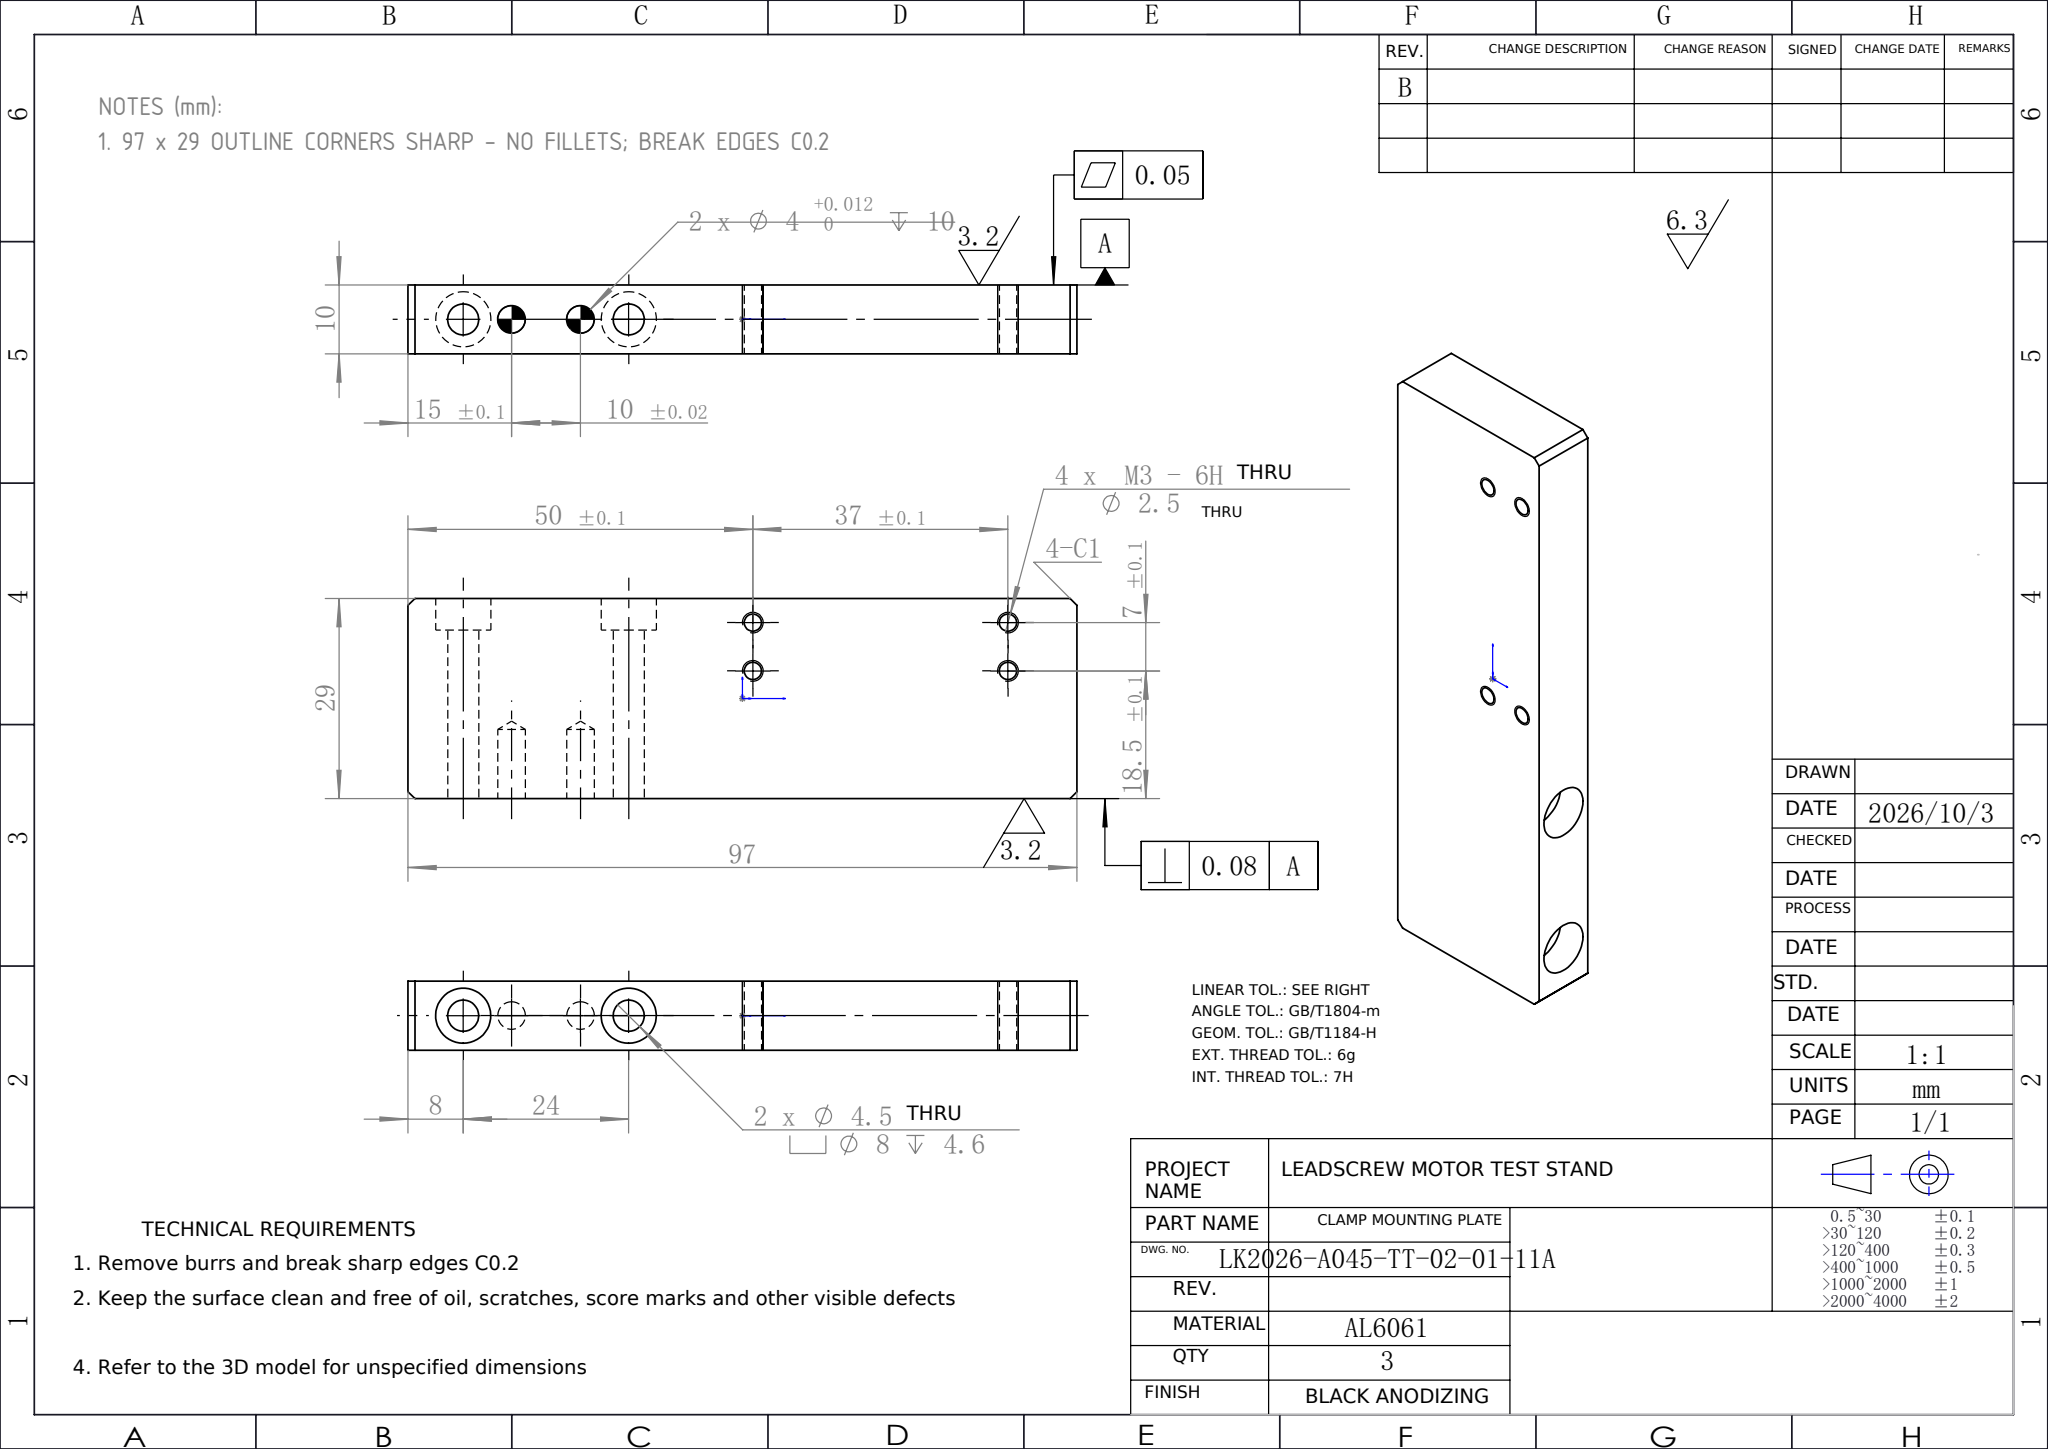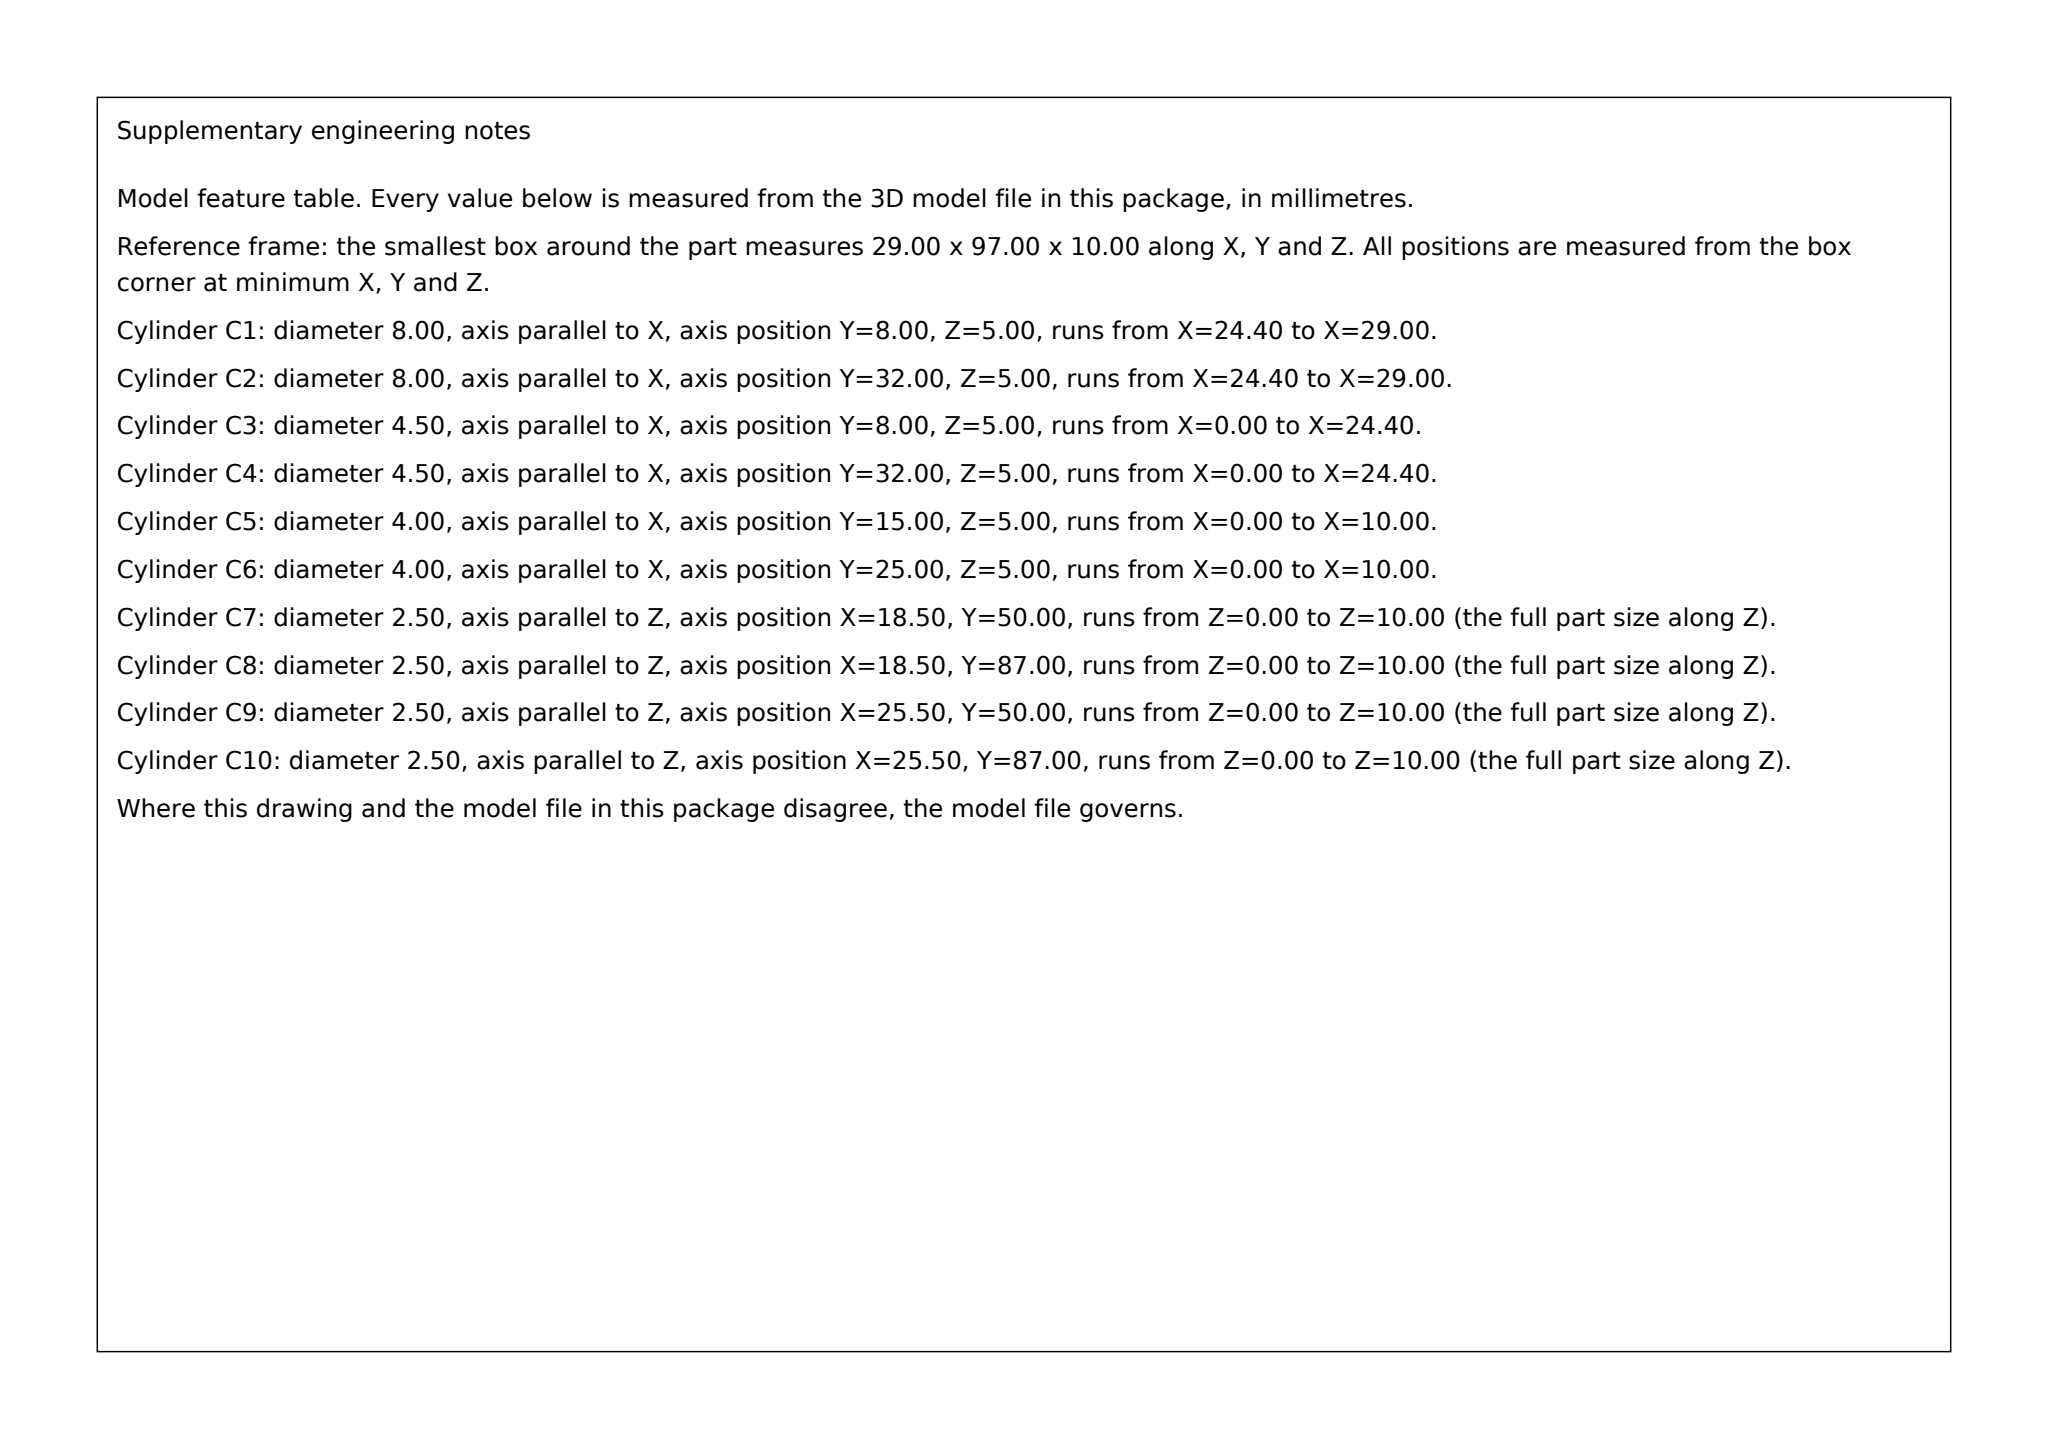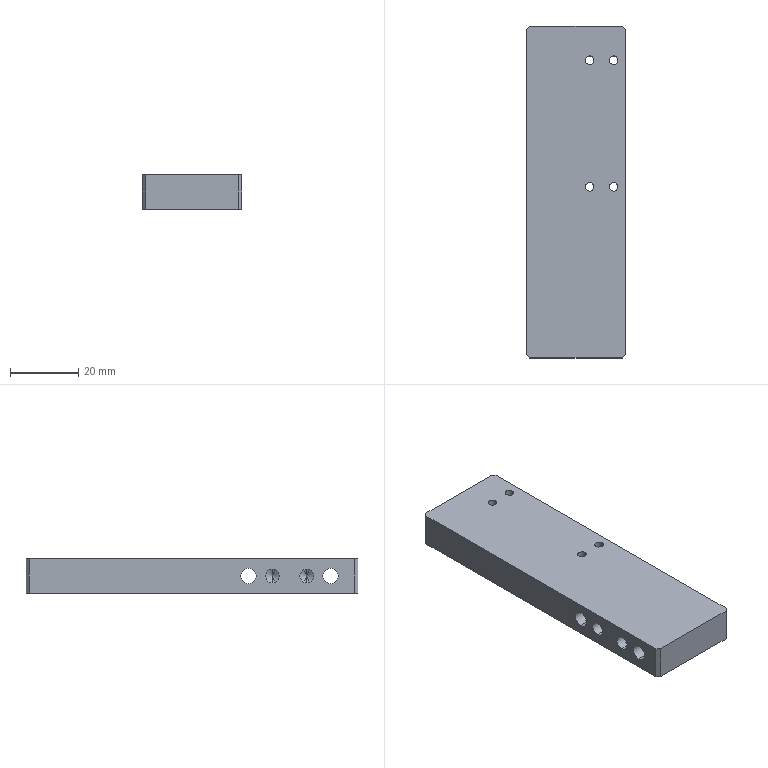Part | SolidWorks | mm | 1 solid | 36 faces | box 29 x 97 x 10 mm | volume 26414 mm3 | cylinder 20 | plane 12 | cone 4 | commonest cylinder face diameters 2.5 x8 4 x4 8 x4 4.5 x4
Drawing notes:
97 x 29 OUTLINE CORNERS SHARP - NO FILLETS; BREAK EDGES C0.2 | from the solid: fillet_radii: []; planar faces x=0/29.0, y=0/97.0; bbox 29.0 x 97.0 x 10.0
build123d program:
from build123d import *

# Parameters (mm, degrees)
SKETCH1_W                                       = 29
SKETCH1_H                                       = 97
BOSS_EXTRUDE1_DEPTH                             = 5
M4_HEX_SOCKET_HEAD_CAP_SCREW_CBORE1_D           = 4.5
M4_HEX_SOCKET_HEAD_CAP_SCREW_CBORE1_CBORE_D     = 8
M4_HEX_SOCKET_HEAD_CAP_SCREW_CBORE1_CBORE_DEPTH = 4.6
F_4_0MM_DOWEL_PIN_HOLE1_D                       = 4
F_4_0MM_DOWEL_PIN_HOLE1_DEPTH                   = 10
F_4_0MM_DOWEL_PIN_HOLE1_TIP                     = 1.202
M3_TAPPED_HOLE1_D                               = 2.5
CHAMFER1_SIZE                                   = 1


with BuildPart() as part:
    # Sketch1 → Boss-Extrude1 (new, symmetric)
    with BuildSketch(Plane.XY):
        Rectangle(SKETCH1_W, SKETCH1_H)
    extrude(amount=BOSS_EXTRUDE1_DEPTH, both=True)

    # M4 Hex Socket Head Cap Screw CBORE1 (through all)
    with Locations(Plane(origin=(14.5, 0, 0), x_dir=(0, 0, -1), z_dir=(1, 0, 0))):
        with Locations((0, -40.5), (0, -16.5)):
            CounterBoreHole(M4_HEX_SOCKET_HEAD_CAP_SCREW_CBORE1_D / 2, M4_HEX_SOCKET_HEAD_CAP_SCREW_CBORE1_CBORE_D / 2, M4_HEX_SOCKET_HEAD_CAP_SCREW_CBORE1_CBORE_DEPTH)

    # 4.0mm Dowel Pin Hole1
    with Locations(Plane.ZY.offset(14.5)):
        with Locations((0, -23.5), (0, -33.5)):
            Hole(F_4_0MM_DOWEL_PIN_HOLE1_D / 2, depth=F_4_0MM_DOWEL_PIN_HOLE1_DEPTH)
            with Locations((0, 0, -(F_4_0MM_DOWEL_PIN_HOLE1_DEPTH + F_4_0MM_DOWEL_PIN_HOLE1_TIP / 2))):  # 118° drill point
                Cone(0, F_4_0MM_DOWEL_PIN_HOLE1_D / 2, F_4_0MM_DOWEL_PIN_HOLE1_TIP, mode=Mode.SUBTRACT)

    # M3 Tapped Hole1 (through all)
    with Locations(Plane.XY.offset(5)):
        with Locations((4, 1.5), (11, 1.5), (11, 38.5), (4, 38.5)):
            Hole(M3_TAPPED_HOLE1_D / 2)

    # Chamfer1
    chamfer1_edges = [part.edges().sort_by_distance(p)[0] for p in [
        (14.5, -48.5, 0),
        (-14.5, -48.5, 0),
        (-14.5, 48.5, 0),
        (14.5, 48.5, 0),
    ]]
    chamfer(chamfer1_edges, length=CHAMFER1_SIZE)


solid = part.part